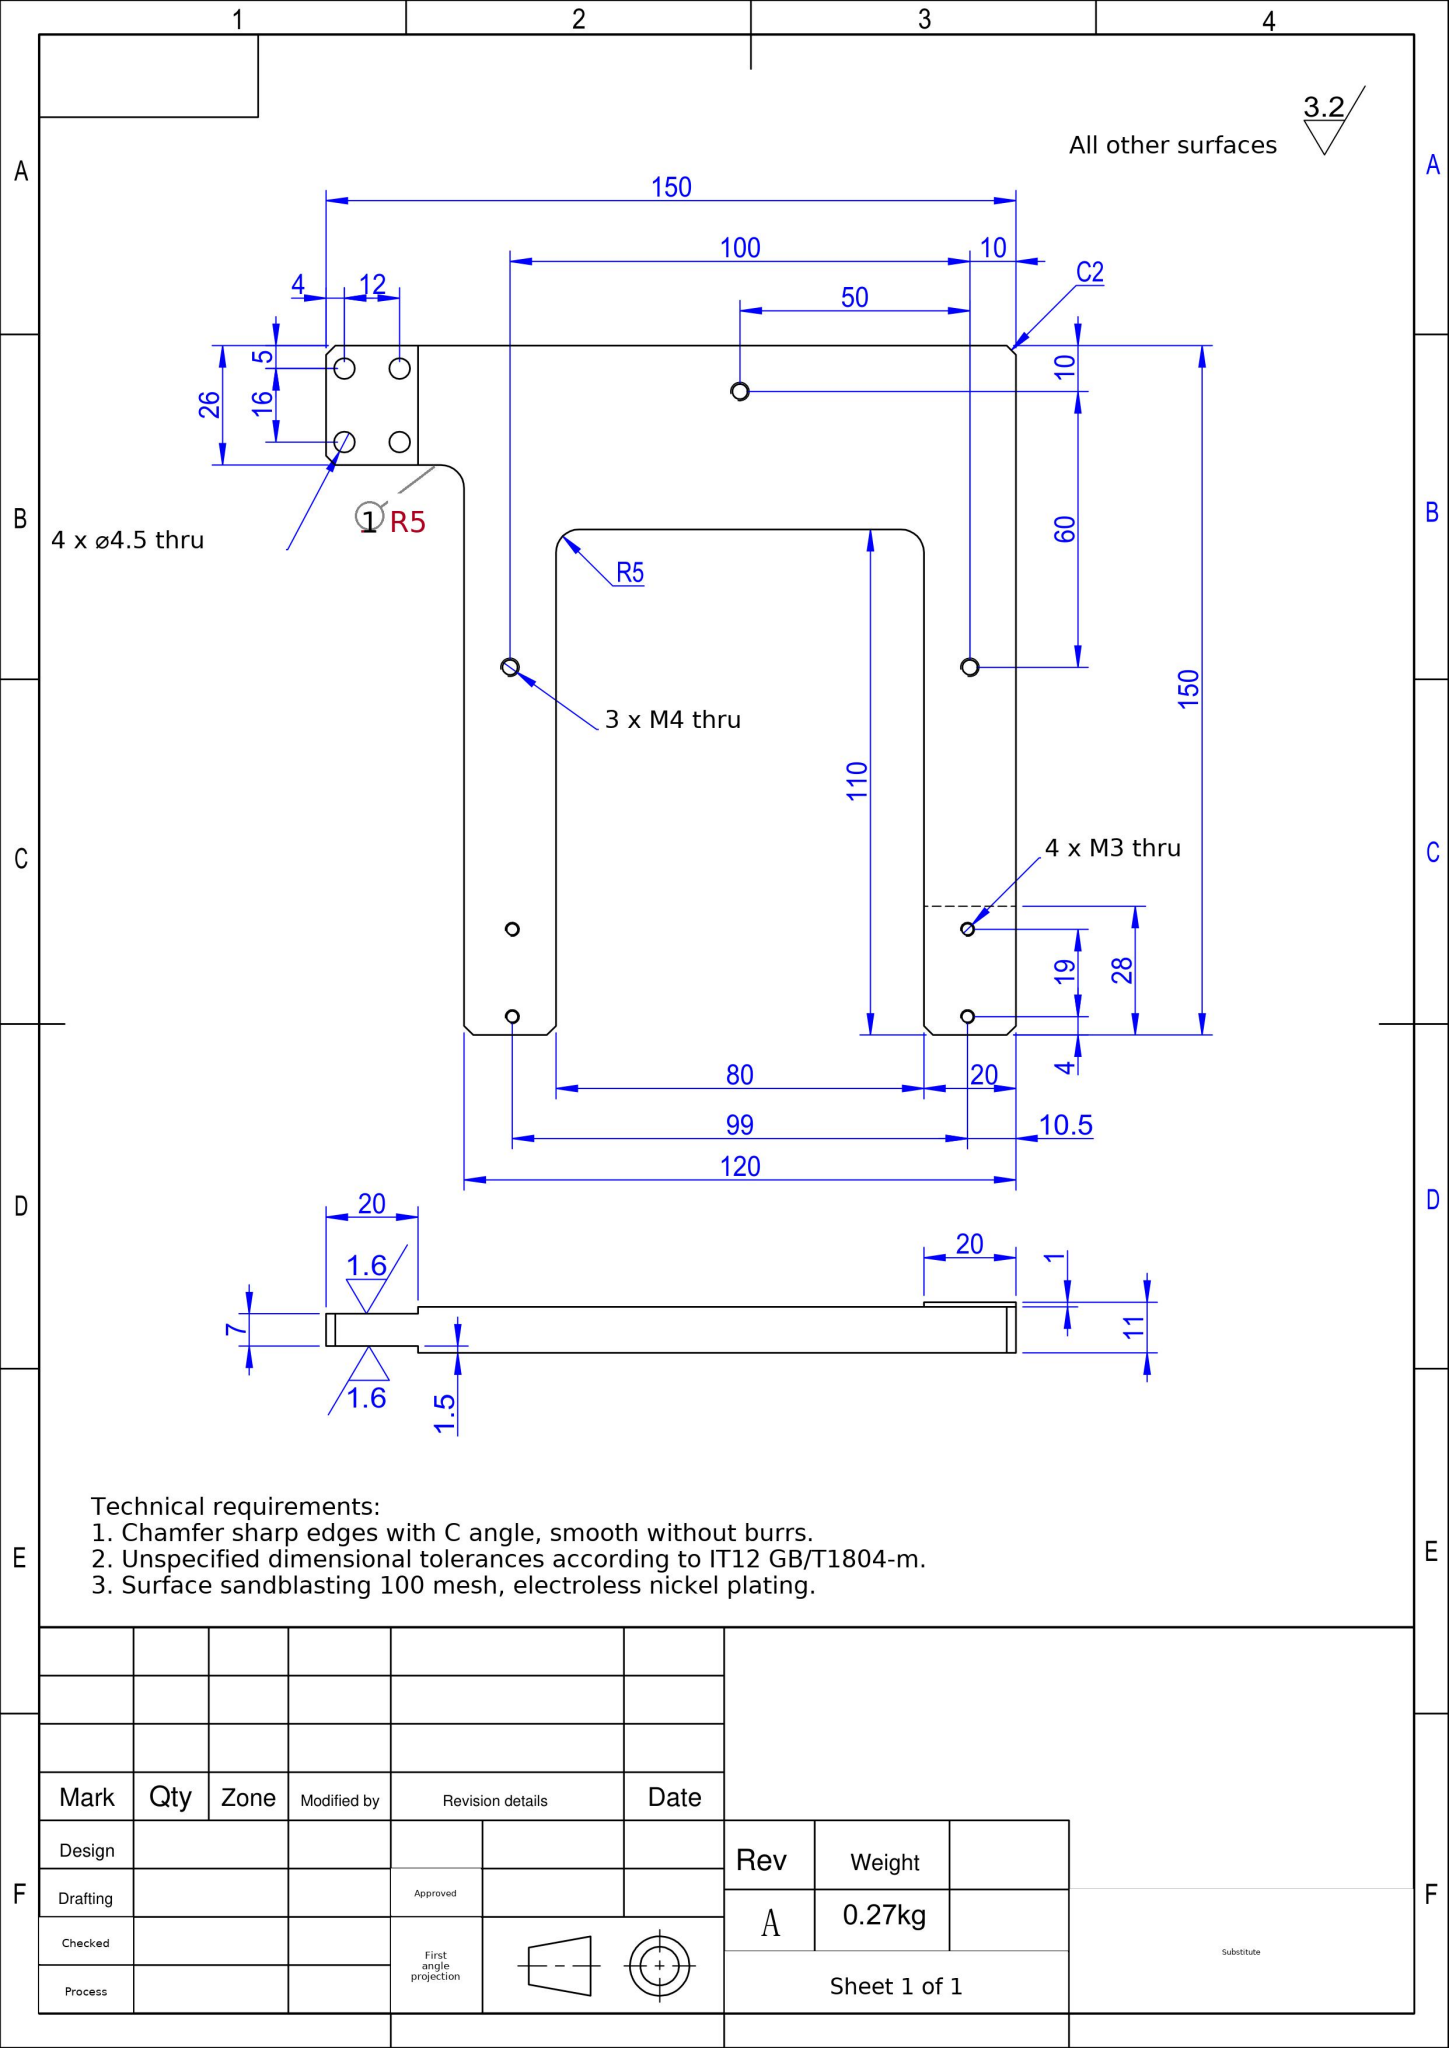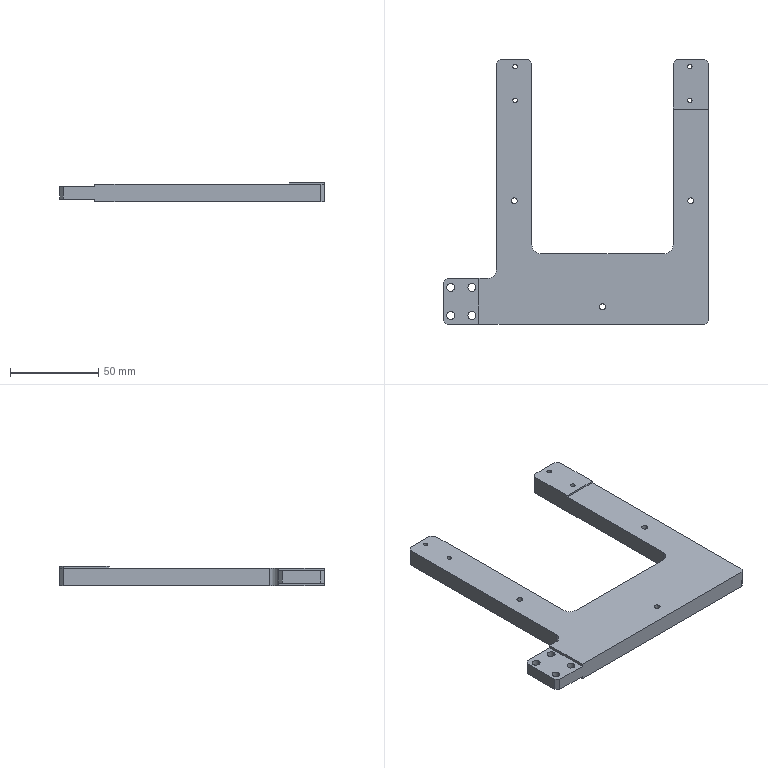Part | SolidWorks | mm | 1 solid | 50 faces | box 150 x 150 x 11 mm | volume 97921 mm3 | cylinder 25 | plane 25 | commonest cylinder face diameters 2.5 x8 4.5 x8 3.3 x6 10 x3
build123d program:
from build123d import *

# Parameters (mm, degrees)
SKETCH1_W            = 120
SKETCH1_H            = 150
BOSS_EXTRUDE1_DEPTH  = 5
SKETCH2_W            = 80
SKETCH2_H            = 110
CUT_EXTRUDE1_DEPTH   = 10
SKETCH8_W            = 20
SKETCH8_H            = 28
BOSS_EXTRUDE2_DEPTH  = 1
SKETCH16_W           = 30
SKETCH16_H           = 26
BOSS_EXTRUDE3_DEPTH  = 10
CHAMFER1_SIZE        = 2
FILLET1_R            = 5
M4_CLEARANCE_HOLE1_D = 4.5
M3_TAPPED_HOLE2_D    = 2.5
M4_TAPPED_HOLE1_D    = 3.3
SKETCH17_W           = 20
SKETCH17_H           = 26
CUT_EXTRUDE4_DEPTH   = 1.5


with BuildPart() as part:
    # Sketch1 → Boss-Extrude1 (new, symmetric)
    with BuildSketch(Plane.XY):
        Rectangle(SKETCH1_W, SKETCH1_H)
    extrude(amount=BOSS_EXTRUDE1_DEPTH, both=True)

    # Sketch2 → Cut-Extrude1 (cut)
    with BuildSketch(Plane.XY.offset(5)):
        with Locations((0, 20)):
            Rectangle(SKETCH2_W, SKETCH2_H)
    extrude(amount=-CUT_EXTRUDE1_DEPTH, mode=Mode.SUBTRACT)

    # Sketch8 → Boss-Extrude2 (add)
    with BuildSketch(Plane.XY.offset(5)):
        with Locations((50, 61)):
            Rectangle(SKETCH8_W, SKETCH8_H)
    extrude(amount=BOSS_EXTRUDE2_DEPTH)

    # Sketch16 → Boss-Extrude3 (add)
    with BuildSketch(Plane.XY.offset(5)):
        with Locations((-75, -62)):
            Rectangle(SKETCH16_W, SKETCH16_H)
    extrude(amount=-BOSS_EXTRUDE3_DEPTH)

    # Chamfer1
    chamfer1_edges = [part.edges().sort_by_distance(p)[0] for p in [
        (60, -75, 0),
        (-60, 75, 0),
        (-40, 75, 0),
        (60, 75, 0.5),
        (40, 75, 0.5),
        (-90, -75, 0),
        (-90, -49, 0),
    ]]
    chamfer(chamfer1_edges, length=CHAMFER1_SIZE)

    # Fillet1
    fillet1_edges = [part.edges().sort_by_distance(p)[0] for p in [
        (40, -35, 0),
        (-40, -35, 0),
        (-60, -49, 0),
    ]]
    fillet(fillet1_edges, radius=FILLET1_R)

    # M4 Clearance Hole1 (through all)
    with Locations(Plane.XY.offset(5)):
        with Locations((-74, -54), (-86, -70), (-74, -70), (-86, -54)):
            Hole(M4_CLEARANCE_HOLE1_D / 2)

    # M3 Tapped Hole2 (through all)
    with Locations(Plane(origin=(0, 0, -5), x_dir=(-1, 0, 0), z_dir=(0, 0, -1))):
        with Locations((49.5, 52), (49.5, 71)):
            m3_tapped_hole2 = Hole(M3_TAPPED_HOLE2_D / 2)

    # Mirror2: M3 Tapped Hole2 across plane
    add(m3_tapped_hole2.mirror(Plane(origin=(0, 0, 0), x_dir=(0, 0, 1), z_dir=(1, 0, 0))), mode=Mode.SUBTRACT)

    # M4 Tapped Hole1 (through all)
    with Locations(Plane.XY.offset(5)):
        with Locations((0, -65), (-50, -5), (50, -5)):
            Hole(M4_TAPPED_HOLE1_D / 2)

    # Sketch17 → Cut-Extrude4 (cut)
    with BuildSketch(Plane.XY.offset(5)):
        with Locations((-80, -62)):
            Rectangle(SKETCH17_W, SKETCH17_H)
    cut_extrude4 = extrude(amount=-CUT_EXTRUDE4_DEPTH, mode=Mode.SUBTRACT)

    # Mirror5: Cut-Extrude4 across plane
    add(cut_extrude4.mirror(Plane.XY), mode=Mode.SUBTRACT)


solid = part.part